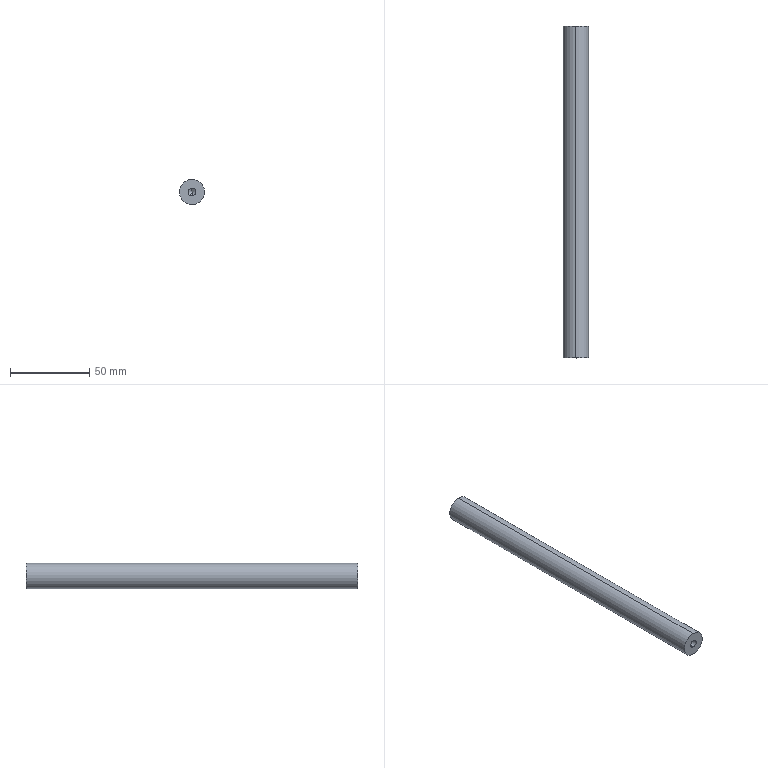Component | SolidWorks | 75-02-13StirringFixedOpticalAxis-1 | 1 solid | 12 faces | box 16 x 210 x 16 mm | volume 41614 mm3 | cylinder 6 | cone 4 | plane 2 | commonest cylinder face diameters 5 x4 16 x2 | material A3 Steel
build123d program:
from build123d import *

# Parameters (mm, degrees)
SKETCH1_R                       = 8
BOSS_EXTRUDE1_DEPTH             = 105
M6_TAPPED_HOLE1_D               = 5
M6_TAPPED_HOLE1_DEPTH           = 15
M6_TAPPED_HOLE1_TIP             = 1.502
M6_TAPPED_HOLE1_ON_FACE_2_D     = 5
M6_TAPPED_HOLE1_ON_FACE_2_DEPTH = 15
M6_TAPPED_HOLE1_ON_FACE_2_TIP   = 1.502


with BuildPart() as part:
    # Sketch1 → Boss-Extrude1 (new, symmetric)
    with BuildSketch(Plane.XY):
        Circle(SKETCH1_R)
    extrude(amount=BOSS_EXTRUDE1_DEPTH, both=True)

    # M6 Tapped Hole1
    with Locations(Plane.XY.offset(105)):
        with Locations((0, 0)):
            Hole(M6_TAPPED_HOLE1_D / 2, depth=M6_TAPPED_HOLE1_DEPTH)
            with Locations((0, 0, -(M6_TAPPED_HOLE1_DEPTH + M6_TAPPED_HOLE1_TIP / 2))):  # 118° drill point
                Cone(0, M6_TAPPED_HOLE1_D / 2, M6_TAPPED_HOLE1_TIP, mode=Mode.SUBTRACT)

    # M6 Tapped Hole1 on face 2
    with Locations(Plane(origin=(0, 0, -105), x_dir=(-1, 0, 0), z_dir=(0, 0, -1))):
        with Locations((0, 0)):
            Hole(M6_TAPPED_HOLE1_ON_FACE_2_D / 2, depth=M6_TAPPED_HOLE1_ON_FACE_2_DEPTH)
            with Locations((0, 0, -(M6_TAPPED_HOLE1_ON_FACE_2_DEPTH + M6_TAPPED_HOLE1_ON_FACE_2_TIP / 2))):  # 118° drill point
                Cone(0, M6_TAPPED_HOLE1_ON_FACE_2_D / 2, M6_TAPPED_HOLE1_ON_FACE_2_TIP, mode=Mode.SUBTRACT)


solid = part.part

# Placed as in the assembly
solid = solid.moved(Location((-67.8, 11.867, 29.75), (90, 0, 0)))
STEP:
#1=CARTESIAN_POINT('',(-2.666,4.011,1.073));
#2=VERTEX_POINT('',#1);
#3=CARTESIAN_POINT('',(-2.673,4.011,1.27));
#4=VERTEX_POINT('',#3);
#5=CARTESIAN_POINT('',(-2.669,4.011,1.171));
#6=DIRECTION('',(0.,1.,0.));
#7=DIRECTION('',(-0.03567,0.,0.9994));
#8=AXIS2_PLACEMENT_3D('',#5,#6,#7);
#9=CIRCLE('',#8,0.09843);
#10=EDGE_CURVE('',#2,#4,#9,.T.);
#11=ORIENTED_EDGE('',*,*,#10,.F.);
#12=CARTESIAN_POINT('',(-2.666,4.601,1.073));
#13=VERTEX_POINT('',#12);
#14=CARTESIAN_POINT('',(-2.666,4.601,1.073));
#15=DIRECTION('',(0.,1.,0.));
#16=VECTOR('',#15,39.37);
#17=LINE('',#14,#16);
#18=EDGE_CURVE('',#2,#13,#17,.T.);
#19=ORIENTED_EDGE('',*,*,#18,.T.);
#20=CARTESIAN_POINT('',(-2.673,4.601,1.27));
#21=VERTEX_POINT('',#20);
#22=CARTESIAN_POINT('',(-2.669,4.601,1.171));
#23=DIRECTION('',(0.,1.,0.));
#24=DIRECTION('',(-0.03567,0.,0.9994));
#25=AXIS2_PLACEMENT_3D('',#22,#23,#24);
#26=CIRCLE('',#25,0.09843);
#27=EDGE_CURVE('',#13,#21,#26,.T.);
#28=ORIENTED_EDGE('',*,*,#27,.T.);
#29=CARTESIAN_POINT('',(-2.673,4.601,1.27));
#30=DIRECTION('',(0.,1.,0.));
#31=VECTOR('',#30,39.37);
#32=LINE('',#29,#31);
#33=EDGE_CURVE('',#4,#21,#32,.T.);
#34=ORIENTED_EDGE('',*,*,#33,.F.);
#35=EDGE_LOOP('',(#11,#19,#28,#34));
#36=FACE_OUTER_BOUND('',#35,.T.);
#37=CARTESIAN_POINT('',(-2.669,4.601,1.171));
#38=DIRECTION('',(0.,1.,0.));
#39=DIRECTION('',(-0.03567,0.,0.9994));
#40=AXIS2_PLACEMENT_3D('',#37,#38,#39);
#41=CYLINDRICAL_SURFACE('',#40,0.09843);
#42=ADVANCED_FACE('',(#36),#41,.F.);
#43=CARTESIAN_POINT('',(-2.669,3.951,1.171));
#44=VERTEX_POINT('',#43);
#45=CARTESIAN_POINT('',(-2.673,4.011,1.27));
#46=DIRECTION('',(-0.03058,0.515,0.8566));
#47=VECTOR('',#46,39.37);
#48=LINE('',#45,#47);
#49=EDGE_CURVE('',#44,#4,#48,.T.);
#50=ORIENTED_EDGE('',*,*,#49,.F.);
#51=CARTESIAN_POINT('',(-2.666,4.011,1.073));
#52=DIRECTION('',(0.03058,0.515,-0.8566));
#53=VECTOR('',#52,39.37);
#54=LINE('',#51,#53);
#55=EDGE_CURVE('',#44,#2,#54,.T.);
#56=ORIENTED_EDGE('',*,*,#55,.T.);
#57=ORIENTED_EDGE('',*,*,#10,.T.);
#58=EDGE_LOOP('',(#50,#56,#57));
#59=FACE_OUTER_BOUND('',#58,.T.);
#60=CARTESIAN_POINT('',(-2.669,4.011,1.171));
#61=DIRECTION('',(0.,1.,0.));
#62=DIRECTION('',(-0.03567,0.,0.9994));
#63=AXIS2_PLACEMENT_3D('',#60,#61,#62);
#64=CONICAL_SURFACE('',#63,0.09843,1.03);
#65=ADVANCED_FACE('',(#59),#64,.F.);
#66=CARTESIAN_POINT('',(-2.673,-3.076,1.27));
#67=VERTEX_POINT('',#66);
#68=CARTESIAN_POINT('',(-2.666,-3.076,1.073));
#69=VERTEX_POINT('',#68);
#70=CARTESIAN_POINT('',(-2.669,-3.076,1.171));
#71=DIRECTION('',(0.,-1.,0.));
#72=DIRECTION('',(0.03567,0.,-0.9994));
#73=AXIS2_PLACEMENT_3D('',#70,#71,#72);
#74=CIRCLE('',#73,0.09843);
#75=EDGE_CURVE('',#67,#69,#74,.T.);
#76=ORIENTED_EDGE('',*,*,#75,.F.);
#77=CARTESIAN_POINT('',(-2.673,-3.667,1.27));
#78=VERTEX_POINT('',#77);
#79=CARTESIAN_POINT('',(-2.673,-3.667,1.27));
#80=DIRECTION('',(0.,-1.,0.));
#81=VECTOR('',#80,39.37);
#82=LINE('',#79,#81);
#83=EDGE_CURVE('',#67,#78,#82,.T.);
#84=ORIENTED_EDGE('',*,*,#83,.T.);
#85=CARTESIAN_POINT('',(-2.666,-3.667,1.073));
#86=VERTEX_POINT('',#85);
#87=CARTESIAN_POINT('',(-2.669,-3.667,1.171));
#88=DIRECTION('',(0.,-1.,0.));
#89=DIRECTION('',(0.03567,0.,-0.9994));
#90=AXIS2_PLACEMENT_3D('',#87,#88,#89);
#91=CIRCLE('',#90,0.09843);
#92=EDGE_CURVE('',#78,#86,#91,.T.);
#93=ORIENTED_EDGE('',*,*,#92,.T.);
#94=CARTESIAN_POINT('',(-2.666,-3.667,1.073));
#95=DIRECTION('',(0.,-1.,0.));
#96=VECTOR('',#95,39.37);
#97=LINE('',#94,#96);
#98=EDGE_CURVE('',#69,#86,#97,.T.);
#99=ORIENTED_EDGE('',*,*,#98,.F.);
#100=EDGE_LOOP('',(#76,#84,#93,#99));
#101=FACE_OUTER_BOUND('',#100,.T.);
#102=CARTESIAN_POINT('',(-2.669,-3.667,1.171));
#103=DIRECTION('',(0.,-1.,0.));
#104=DIRECTION('',(0.03567,0.,-0.9994));
#105=AXIS2_PLACEMENT_3D('',#102,#103,#104);
#106=CYLINDRICAL_SURFACE('',#105,0.09843);
#107=ADVANCED_FACE('',(#101),#106,.F.);
#108=CARTESIAN_POINT('',(-2.669,-3.017,1.171));
#109=VERTEX_POINT('',#108);
#110=CARTESIAN_POINT('',(-2.666,-3.076,1.073));
#111=DIRECTION('',(0.03058,-0.515,-0.8566));
#112=VECTOR('',#111,39.37);
#113=LINE('',#110,#112);
#114=EDGE_CURVE('',#109,#69,#113,.T.);
#115=ORIENTED_EDGE('',*,*,#114,.F.);
#116=CARTESIAN_POINT('',(-2.673,-3.076,1.27));
#117=DIRECTION('',(-0.03058,-0.515,0.8566));
#118=VECTOR('',#117,39.37);
#119=LINE('',#116,#118);
#120=EDGE_CURVE('',#109,#67,#119,.T.);
#121=ORIENTED_EDGE('',*,*,#120,.T.);
#122=ORIENTED_EDGE('',*,*,#75,.T.);
#123=EDGE_LOOP('',(#115,#121,#122));
#124=FACE_OUTER_BOUND('',#123,.T.);
#125=CARTESIAN_POINT('',(-2.669,-3.076,1.171));
#126=DIRECTION('',(0.,-1.,0.));
#127=DIRECTION('',(0.03567,0.,-0.9994));
#128=AXIS2_PLACEMENT_3D('',#125,#126,#127);
#129=CONICAL_SURFACE('',#128,0.09843,1.03);
#130=ADVANCED_FACE('',(#124),#129,.F.);
#131=CARTESIAN_POINT('',(-2.681,4.601,1.486));
#132=VERTEX_POINT('',#131);
#133=CARTESIAN_POINT('',(-2.658,4.601,0.8565));
#134=VERTEX_POINT('',#133);
#135=CARTESIAN_POINT('',(-2.669,4.601,1.171));
#136=DIRECTION('',(0.,1.,0.));
#137=DIRECTION('',(-0.03567,0.,0.9994));
#138=AXIS2_PLACEMENT_3D('',#135,#136,#137);
#139=CIRCLE('',#138,0.315);
#140=EDGE_CURVE('',#132,#134,#139,.T.);
#141=ORIENTED_EDGE('',*,*,#140,.F.);
#142=CARTESIAN_POINT('',(-2.681,-3.667,1.486));
#143=VERTEX_POINT('',#142);
#144=CARTESIAN_POINT('',(-2.681,4.601,1.486));
#145=DIRECTION('',(0.,-1.,0.));
#146=VECTOR('',#145,39.37);
#147=LINE('',#144,#146);
#148=EDGE_CURVE('',#132,#143,#147,.T.);
#149=ORIENTED_EDGE('',*,*,#148,.T.);
#150=CARTESIAN_POINT('',(-2.658,-3.667,0.8565));
#151=VERTEX_POINT('',#150);
#152=CARTESIAN_POINT('',(-2.669,-3.667,1.171));
#153=DIRECTION('',(0.,1.,0.));
#154=DIRECTION('',(-0.03567,0.,0.9994));
#155=AXIS2_PLACEMENT_3D('',#152,#153,#154);
#156=CIRCLE('',#155,0.315);
#157=EDGE_CURVE('',#143,#151,#156,.T.);
#158=ORIENTED_EDGE('',*,*,#157,.T.);
#159=CARTESIAN_POINT('',(-2.658,4.601,0.8565));
#160=DIRECTION('',(0.,-1.,0.));
#161=VECTOR('',#160,39.37);
#162=LINE('',#159,#161);
#163=EDGE_CURVE('',#134,#151,#162,.T.);
#164=ORIENTED_EDGE('',*,*,#163,.F.);
#165=EDGE_LOOP('',(#141,#149,#158,#164));
#166=FACE_OUTER_BOUND('',#165,.T.);
#167=CARTESIAN_POINT('',(-2.669,4.601,1.171));
#168=DIRECTION('',(0.,-1.,0.));
#169=DIRECTION('',(0.03567,0.,-0.9994));
#170=AXIS2_PLACEMENT_3D('',#167,#168,#169);
#171=CYLINDRICAL_SURFACE('',#170,0.315);
#172=ADVANCED_FACE('',(#166),#171,.T.);
#173=ORIENTED_EDGE('',*,*,#148,.F.);
#174=CARTESIAN_POINT('',(-2.669,4.601,1.171));
#175=DIRECTION('',(0.,1.,0.));
#176=DIRECTION('',(-0.03567,0.,0.9994));
#177=AXIS2_PLACEMENT_3D('',#174,#175,#176);
#178=CIRCLE('',#177,0.315);
#179=EDGE_CURVE('',#134,#132,#178,.T.);
#180=ORIENTED_EDGE('',*,*,#179,.F.);
#181=ORIENTED_EDGE('',*,*,#163,.T.);
#182=CARTESIAN_POINT('',(-2.669,-3.667,1.171));
#183=DIRECTION('',(0.,1.,0.));
#184=DIRECTION('',(-0.03567,0.,0.9994));
#185=AXIS2_PLACEMENT_3D('',#182,#183,#184);
#186=CIRCLE('',#185,0.315);
#187=EDGE_CURVE('',#151,#143,#186,.T.);
#188=ORIENTED_EDGE('',*,*,#187,.T.);
#189=EDGE_LOOP('',(#173,#180,#181,#188));
#190=FACE_OUTER_BOUND('',#189,.T.);
#191=CARTESIAN_POINT('',(-2.669,4.601,1.171));
#192=DIRECTION('',(0.,-1.,0.));
#193=DIRECTION('',(0.03567,0.,-0.9994));
#194=AXIS2_PLACEMENT_3D('',#191,#192,#193);
#195=CYLINDRICAL_SURFACE('',#194,0.315);
#196=ADVANCED_FACE('',(#190),#195,.T.);
#197=CARTESIAN_POINT('',(-2.669,4.601,1.171));
#198=DIRECTION('',(0.,1.,0.));
#199=DIRECTION('',(-0.03567,0.,0.9994));
#200=AXIS2_PLACEMENT_3D('',#197,#198,#199);
#201=CIRCLE('',#200,0.09843);
#202=EDGE_CURVE('',#21,#13,#201,.T.);
#203=ORIENTED_EDGE('',*,*,#202,.F.);
#204=ORIENTED_EDGE('',*,*,#27,.F.);
#205=EDGE_LOOP('',(#203,#204));
#206=FACE_BOUND('',#205,.T.);
#207=ORIENTED_EDGE('',*,*,#179,.T.);
#208=ORIENTED_EDGE('',*,*,#140,.T.);
#209=EDGE_LOOP('',(#207,#208));
#210=FACE_OUTER_BOUND('',#209,.T.);
#211=CARTESIAN_POINT('',(-2.669,4.601,1.171));
#212=DIRECTION('',(0.,1.,0.));
#213=DIRECTION('',(-0.03567,0.,0.9994));
#214=AXIS2_PLACEMENT_3D('',#211,#212,#213);
#215=PLANE('',#214);
#216=ADVANCED_FACE('',(#206,#210),#215,.T.);
#217=CARTESIAN_POINT('',(-2.669,-3.667,1.171));
#218=DIRECTION('',(0.,-1.,0.));
#219=DIRECTION('',(0.03567,0.,-0.9994));
#220=AXIS2_PLACEMENT_3D('',#217,#218,#219);
#221=CIRCLE('',#220,0.09843);
#222=EDGE_CURVE('',#86,#78,#221,.T.);
#223=ORIENTED_EDGE('',*,*,#222,.F.);
#224=ORIENTED_EDGE('',*,*,#92,.F.);
#225=EDGE_LOOP('',(#223,#224));
#226=FACE_BOUND('',#225,.T.);
#227=ORIENTED_EDGE('',*,*,#187,.F.);
#228=ORIENTED_EDGE('',*,*,#157,.F.);
#229=EDGE_LOOP('',(#227,#228));
#230=FACE_OUTER_BOUND('',#229,.T.);
#231=CARTESIAN_POINT('',(-2.669,-3.667,1.171));
#232=DIRECTION('',(0.,1.,0.));
#233=DIRECTION('',(-0.03567,0.,0.9994));
#234=AXIS2_PLACEMENT_3D('',#231,#232,#233);
#235=PLANE('',#234);
#236=ADVANCED_FACE('',(#226,#230),#235,.F.);
#237=ORIENTED_EDGE('',*,*,#120,.F.);
#238=ORIENTED_EDGE('',*,*,#114,.T.);
#239=CARTESIAN_POINT('',(-2.669,-3.076,1.171));
#240=DIRECTION('',(0.,-1.,0.));
#241=DIRECTION('',(0.03567,0.,-0.9994));
#242=AXIS2_PLACEMENT_3D('',#239,#240,#241);
#243=CIRCLE('',#242,0.09843);
#244=EDGE_CURVE('',#69,#67,#243,.T.);
#245=ORIENTED_EDGE('',*,*,#244,.T.);
#246=EDGE_LOOP('',(#237,#238,#245));
#247=FACE_OUTER_BOUND('',#246,.T.);
#248=CARTESIAN_POINT('',(-2.669,-3.076,1.171));
#249=DIRECTION('',(0.,-1.,0.));
#250=DIRECTION('',(0.03567,0.,-0.9994));
#251=AXIS2_PLACEMENT_3D('',#248,#249,#250);
#252=CONICAL_SURFACE('',#251,0.09843,1.03);
#253=ADVANCED_FACE('',(#247),#252,.F.);
#254=ORIENTED_EDGE('',*,*,#83,.F.);
#255=ORIENTED_EDGE('',*,*,#244,.F.);
#256=ORIENTED_EDGE('',*,*,#98,.T.);
#257=ORIENTED_EDGE('',*,*,#222,.T.);
#258=EDGE_LOOP('',(#254,#255,#256,#257));
#259=FACE_OUTER_BOUND('',#258,.T.);
#260=CARTESIAN_POINT('',(-2.669,-3.667,1.171));
#261=DIRECTION('',(0.,-1.,0.));
#262=DIRECTION('',(0.03567,0.,-0.9994));
#263=AXIS2_PLACEMENT_3D('',#260,#261,#262);
#264=CYLINDRICAL_SURFACE('',#263,0.09843);
#265=ADVANCED_FACE('',(#259),#264,.F.);
#266=ORIENTED_EDGE('',*,*,#55,.F.);
#267=ORIENTED_EDGE('',*,*,#49,.T.);
#268=CARTESIAN_POINT('',(-2.669,4.011,1.171));
#269=DIRECTION('',(0.,1.,0.));
#270=DIRECTION('',(-0.03567,0.,0.9994));
#271=AXIS2_PLACEMENT_3D('',#268,#269,#270);
#272=CIRCLE('',#271,0.09843);
#273=EDGE_CURVE('',#4,#2,#272,.T.);
#274=ORIENTED_EDGE('',*,*,#273,.T.);
#275=EDGE_LOOP('',(#266,#267,#274));
#276=FACE_OUTER_BOUND('',#275,.T.);
#277=CARTESIAN_POINT('',(-2.669,4.011,1.171));
#278=DIRECTION('',(0.,1.,0.));
#279=DIRECTION('',(-0.03567,0.,0.9994));
#280=AXIS2_PLACEMENT_3D('',#277,#278,#279);
#281=CONICAL_SURFACE('',#280,0.09843,1.03);
#282=ADVANCED_FACE('',(#276),#281,.F.);
#283=ORIENTED_EDGE('',*,*,#18,.F.);
#284=ORIENTED_EDGE('',*,*,#273,.F.);
#285=ORIENTED_EDGE('',*,*,#33,.T.);
#286=ORIENTED_EDGE('',*,*,#202,.T.);
#287=EDGE_LOOP('',(#283,#284,#285,#286));
#288=FACE_OUTER_BOUND('',#287,.T.);
#289=CARTESIAN_POINT('',(-2.669,4.601,1.171));
#290=DIRECTION('',(0.,1.,0.));
#291=DIRECTION('',(-0.03567,0.,0.9994));
#292=AXIS2_PLACEMENT_3D('',#289,#290,#291);
#293=CYLINDRICAL_SURFACE('',#292,0.09843);
#294=ADVANCED_FACE('',(#288),#293,.F.);
#295=CLOSED_SHELL('',(#42,#65,#107,#130,#172,#196,#216,#236,#253,#265,#282,#294));
#296=MANIFOLD_SOLID_BREP('',#295);
#297=CARTESIAN_POINT('',(0.,0.,0.));
#298=DIRECTION('',(0.,0.,1.));
#299=DIRECTION('',(1.,0.,0.));
#300=AXIS2_PLACEMENT_3D('',#297,#298,#299);
#301=(LENGTH_UNIT()NAMED_UNIT(*)SI_UNIT($,.METRE.));
#302=LENGTH_MEASURE_WITH_UNIT(LENGTH_MEASURE(0.0254),#301);
#303=DIMENSIONAL_EXPONENTS(1.,0.,0.,0.,0.,0.,0.);
#304=(CONVERSION_BASED_UNIT('',#302)LENGTH_UNIT()NAMED_UNIT(#303));
#305=UNCERTAINTY_MEASURE_WITH_UNIT(LENGTH_MEASURE(0.00001),#304,'','');
#306=(NAMED_UNIT(*)PLANE_ANGLE_UNIT()SI_UNIT($,.RADIAN.));
#307=(NAMED_UNIT(*)SI_UNIT($,.STERADIAN.)SOLID_ANGLE_UNIT());
#308=(GEOMETRIC_REPRESENTATION_CONTEXT(3)GLOBAL_UNCERTAINTY_ASSIGNED_CONTEXT((#305))GLOBAL_UNIT_ASSIGNED_CONTEXT((#304,#306,#307))REPRESENTATION_CONTEXT('',''));
#309=ADVANCED_BREP_SHAPE_REPRESENTATION('',(#296,#300),#308);
#310=COLOUR_RGB('',0.7922,0.8196,0.9333);
#311=FILL_AREA_STYLE_COLOUR('',#310);
#312=FILL_AREA_STYLE('',(#311));
#313=SURFACE_STYLE_FILL_AREA(#312);
#314=SURFACE_SIDE_STYLE('',(#313));
#315=SURFACE_STYLE_USAGE(.BOTH.,#314);
#316=PRESENTATION_STYLE_ASSIGNMENT((#315));
#317=STYLED_ITEM('',(#316),#296);
#318=(LENGTH_UNIT()NAMED_UNIT(*)SI_UNIT($,.METRE.));
#319=LENGTH_MEASURE_WITH_UNIT(LENGTH_MEASURE(0.0254),#318);
#320=DIMENSIONAL_EXPONENTS(1.,0.,0.,0.,0.,0.,0.);
#321=(CONVERSION_BASED_UNIT('',#319)LENGTH_UNIT()NAMED_UNIT(#320));
#322=UNCERTAINTY_MEASURE_WITH_UNIT(LENGTH_MEASURE(0.00001),#321,'','');
#323=(NAMED_UNIT(*)PLANE_ANGLE_UNIT()SI_UNIT($,.RADIAN.));
#324=(NAMED_UNIT(*)SI_UNIT($,.STERADIAN.)SOLID_ANGLE_UNIT());
#325=(GEOMETRIC_REPRESENTATION_CONTEXT(3)GLOBAL_UNCERTAINTY_ASSIGNED_CONTEXT((#322))GLOBAL_UNIT_ASSIGNED_CONTEXT((#321,#323,#324))REPRESENTATION_CONTEXT('',''));
#326=MECHANICAL_DESIGN_GEOMETRIC_PRESENTATION_REPRESENTATION('',(#317),#325);
#327=PRESENTATION_LAYER_ASSIGNMENT('','',(#317));